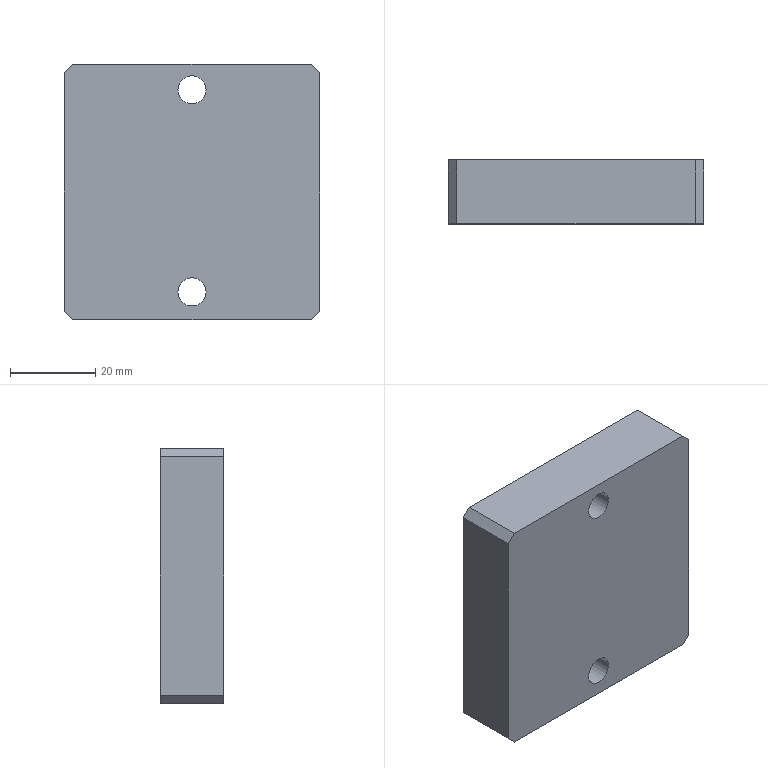Component | SolidWorks | CHEN123-AA-08-1 | 1 solid | 20 faces | box 60 x 15 x 60 mm | volume 52075 mm3 | plane 12 | cylinder 8 | commonest cylinder face diameters 11 x4 6.6 x4
build123d program:
from build123d import *

# Parameters (mm, degrees)
SKETCH1_W                                       = 60
SKETCH1_H                                       = 60
BOSS_EXTRUDE1_DEPTH                             = 15
CHAMFER1_SIZE                                   = 2
M6_HEX_SOCKET_HEAD_CAP_SCREW_CBORE1_D           = 6.6
M6_HEX_SOCKET_HEAD_CAP_SCREW_CBORE1_CBORE_D     = 11
M6_HEX_SOCKET_HEAD_CAP_SCREW_CBORE1_CBORE_DEPTH = 6.4


with BuildPart() as part:
    # Sketch1 → Boss-Extrude1 (new body)
    with BuildSketch(Plane.XY):
        Rectangle(SKETCH1_W, SKETCH1_H)
    extrude(amount=BOSS_EXTRUDE1_DEPTH)

    # Chamfer1
    chamfer1_edges = [part.edges().sort_by_distance(p)[0] for p in [
        (30, -30, 7.5),
        (-30, -30, 7.5),
        (-30, 30, 7.5),
        (30, 30, 7.5),
    ]]
    chamfer(chamfer1_edges, length=CHAMFER1_SIZE)

    # M6 Hex Socket Head Cap Screw CBORE1 (through all)
    with Locations(Plane.XY.offset(15)):
        with Locations((0, 23.473), (0, -23.997)):
            CounterBoreHole(M6_HEX_SOCKET_HEAD_CAP_SCREW_CBORE1_D / 2, M6_HEX_SOCKET_HEAD_CAP_SCREW_CBORE1_CBORE_D / 2, M6_HEX_SOCKET_HEAD_CAP_SCREW_CBORE1_CBORE_DEPTH)


solid = part.part

# Placed as in the assembly
solid = solid.moved(Location((-0.0005, -150.999, -97), (-90, 0, 0)))
STEP:
#1=CARTESIAN_POINT('',(-0.2166,-5.606,-4.743));
#2=VERTEX_POINT('',#1);
#3=CARTESIAN_POINT('',(0.2165,-5.606,-4.743));
#4=VERTEX_POINT('',#3);
#5=CARTESIAN_POINT('',(-0.00001969,-5.606,-4.743));
#6=DIRECTION('',(0.,1.,0.));
#7=DIRECTION('',(1.,0.,0.));
#8=AXIS2_PLACEMENT_3D('',#5,#6,#7);
#9=CIRCLE('',#8,0.2165);
#10=EDGE_CURVE('',#2,#4,#9,.T.);
#11=ORIENTED_EDGE('',*,*,#10,.F.);
#12=CARTESIAN_POINT('',(-0.2166,-5.354,-4.743));
#13=VERTEX_POINT('',#12);
#14=CARTESIAN_POINT('',(-0.2166,-5.354,-4.743));
#15=DIRECTION('',(0.,1.,0.));
#16=VECTOR('',#15,39.37);
#17=LINE('',#14,#16);
#18=EDGE_CURVE('',#2,#13,#17,.T.);
#19=ORIENTED_EDGE('',*,*,#18,.T.);
#20=CARTESIAN_POINT('',(0.2165,-5.354,-4.743));
#21=VERTEX_POINT('',#20);
#22=CARTESIAN_POINT('',(-0.00001969,-5.354,-4.743));
#23=DIRECTION('',(0.,1.,0.));
#24=DIRECTION('',(1.,0.,0.));
#25=AXIS2_PLACEMENT_3D('',#22,#23,#24);
#26=CIRCLE('',#25,0.2165);
#27=EDGE_CURVE('',#13,#21,#26,.T.);
#28=ORIENTED_EDGE('',*,*,#27,.T.);
#29=CARTESIAN_POINT('',(0.2165,-5.354,-4.743));
#30=DIRECTION('',(0.,1.,0.));
#31=VECTOR('',#30,39.37);
#32=LINE('',#29,#31);
#33=EDGE_CURVE('',#4,#21,#32,.T.);
#34=ORIENTED_EDGE('',*,*,#33,.F.);
#35=EDGE_LOOP('',(#11,#19,#28,#34));
#36=FACE_OUTER_BOUND('',#35,.T.);
#37=CARTESIAN_POINT('',(-0.00001969,-5.354,-4.743));
#38=DIRECTION('',(0.,1.,0.));
#39=DIRECTION('',(1.,0.,0.));
#40=AXIS2_PLACEMENT_3D('',#37,#38,#39);
#41=CYLINDRICAL_SURFACE('',#40,0.2165);
#42=ADVANCED_FACE('',(#36),#41,.F.);
#43=CARTESIAN_POINT('',(-0.1299,-5.945,-4.743));
#44=VERTEX_POINT('',#43);
#45=CARTESIAN_POINT('',(0.1299,-5.945,-4.743));
#46=VERTEX_POINT('',#45);
#47=CARTESIAN_POINT('',(-0.00001969,-5.945,-4.743));
#48=DIRECTION('',(0.,1.,0.));
#49=DIRECTION('',(1.,0.,0.));
#50=AXIS2_PLACEMENT_3D('',#47,#48,#49);
#51=CIRCLE('',#50,0.1299);
#52=EDGE_CURVE('',#44,#46,#51,.T.);
#53=ORIENTED_EDGE('',*,*,#52,.F.);
#54=CARTESIAN_POINT('',(-0.1299,-5.606,-4.743));
#55=VERTEX_POINT('',#54);
#56=CARTESIAN_POINT('',(-0.1299,-5.354,-4.743));
#57=DIRECTION('',(0.,1.,0.));
#58=VECTOR('',#57,39.37);
#59=LINE('',#56,#58);
#60=EDGE_CURVE('',#44,#55,#59,.T.);
#61=ORIENTED_EDGE('',*,*,#60,.T.);
#62=CARTESIAN_POINT('',(0.1299,-5.606,-4.743));
#63=VERTEX_POINT('',#62);
#64=CARTESIAN_POINT('',(-0.00001969,-5.606,-4.743));
#65=DIRECTION('',(0.,1.,0.));
#66=DIRECTION('',(1.,0.,0.));
#67=AXIS2_PLACEMENT_3D('',#64,#65,#66);
#68=CIRCLE('',#67,0.1299);
#69=EDGE_CURVE('',#55,#63,#68,.T.);
#70=ORIENTED_EDGE('',*,*,#69,.T.);
#71=CARTESIAN_POINT('',(0.1299,-5.354,-4.743));
#72=DIRECTION('',(0.,1.,0.));
#73=VECTOR('',#72,39.37);
#74=LINE('',#71,#73);
#75=EDGE_CURVE('',#46,#63,#74,.T.);
#76=ORIENTED_EDGE('',*,*,#75,.F.);
#77=EDGE_LOOP('',(#53,#61,#70,#76));
#78=FACE_OUTER_BOUND('',#77,.T.);
#79=CARTESIAN_POINT('',(-0.00001969,-5.354,-4.743));
#80=DIRECTION('',(0.,1.,0.));
#81=DIRECTION('',(1.,0.,0.));
#82=AXIS2_PLACEMENT_3D('',#79,#80,#81);
#83=CYLINDRICAL_SURFACE('',#82,0.1299);
#84=ADVANCED_FACE('',(#78),#83,.F.);
#85=CARTESIAN_POINT('',(-0.2166,-5.606,-2.874));
#86=VERTEX_POINT('',#85);
#87=CARTESIAN_POINT('',(0.2165,-5.606,-2.874));
#88=VERTEX_POINT('',#87);
#89=CARTESIAN_POINT('',(-0.00001969,-5.606,-2.874));
#90=DIRECTION('',(0.,1.,0.));
#91=DIRECTION('',(1.,0.,0.));
#92=AXIS2_PLACEMENT_3D('',#89,#90,#91);
#93=CIRCLE('',#92,0.2165);
#94=EDGE_CURVE('',#86,#88,#93,.T.);
#95=ORIENTED_EDGE('',*,*,#94,.F.);
#96=CARTESIAN_POINT('',(-0.2166,-5.354,-2.874));
#97=VERTEX_POINT('',#96);
#98=CARTESIAN_POINT('',(-0.2166,-5.354,-2.874));
#99=DIRECTION('',(0.,1.,0.));
#100=VECTOR('',#99,39.37);
#101=LINE('',#98,#100);
#102=EDGE_CURVE('',#86,#97,#101,.T.);
#103=ORIENTED_EDGE('',*,*,#102,.T.);
#104=CARTESIAN_POINT('',(0.2165,-5.354,-2.874));
#105=VERTEX_POINT('',#104);
#106=CARTESIAN_POINT('',(-0.00001969,-5.354,-2.874));
#107=DIRECTION('',(0.,1.,0.));
#108=DIRECTION('',(1.,0.,0.));
#109=AXIS2_PLACEMENT_3D('',#106,#107,#108);
#110=CIRCLE('',#109,0.2165);
#111=EDGE_CURVE('',#97,#105,#110,.T.);
#112=ORIENTED_EDGE('',*,*,#111,.T.);
#113=CARTESIAN_POINT('',(0.2165,-5.354,-2.874));
#114=DIRECTION('',(0.,1.,0.));
#115=VECTOR('',#114,39.37);
#116=LINE('',#113,#115);
#117=EDGE_CURVE('',#88,#105,#116,.T.);
#118=ORIENTED_EDGE('',*,*,#117,.F.);
#119=EDGE_LOOP('',(#95,#103,#112,#118));
#120=FACE_OUTER_BOUND('',#119,.T.);
#121=CARTESIAN_POINT('',(-0.00001969,-5.354,-2.874));
#122=DIRECTION('',(0.,1.,0.));
#123=DIRECTION('',(1.,0.,0.));
#124=AXIS2_PLACEMENT_3D('',#121,#122,#123);
#125=CYLINDRICAL_SURFACE('',#124,0.2165);
#126=ADVANCED_FACE('',(#120),#125,.F.);
#127=CARTESIAN_POINT('',(-0.1299,-5.945,-2.874));
#128=VERTEX_POINT('',#127);
#129=CARTESIAN_POINT('',(0.1299,-5.945,-2.874));
#130=VERTEX_POINT('',#129);
#131=CARTESIAN_POINT('',(-0.00001969,-5.945,-2.874));
#132=DIRECTION('',(0.,1.,0.));
#133=DIRECTION('',(1.,0.,0.));
#134=AXIS2_PLACEMENT_3D('',#131,#132,#133);
#135=CIRCLE('',#134,0.1299);
#136=EDGE_CURVE('',#128,#130,#135,.T.);
#137=ORIENTED_EDGE('',*,*,#136,.F.);
#138=CARTESIAN_POINT('',(-0.1299,-5.606,-2.874));
#139=VERTEX_POINT('',#138);
#140=CARTESIAN_POINT('',(-0.1299,-5.354,-2.874));
#141=DIRECTION('',(0.,1.,0.));
#142=VECTOR('',#141,39.37);
#143=LINE('',#140,#142);
#144=EDGE_CURVE('',#128,#139,#143,.T.);
#145=ORIENTED_EDGE('',*,*,#144,.T.);
#146=CARTESIAN_POINT('',(0.1299,-5.606,-2.874));
#147=VERTEX_POINT('',#146);
#148=CARTESIAN_POINT('',(-0.00001969,-5.606,-2.874));
#149=DIRECTION('',(0.,1.,0.));
#150=DIRECTION('',(1.,0.,0.));
#151=AXIS2_PLACEMENT_3D('',#148,#149,#150);
#152=CIRCLE('',#151,0.1299);
#153=EDGE_CURVE('',#139,#147,#152,.T.);
#154=ORIENTED_EDGE('',*,*,#153,.T.);
#155=CARTESIAN_POINT('',(0.1299,-5.354,-2.874));
#156=DIRECTION('',(0.,1.,0.));
#157=VECTOR('',#156,39.37);
#158=LINE('',#155,#157);
#159=EDGE_CURVE('',#130,#147,#158,.T.);
#160=ORIENTED_EDGE('',*,*,#159,.F.);
#161=EDGE_LOOP('',(#137,#145,#154,#160));
#162=FACE_OUTER_BOUND('',#161,.T.);
#163=CARTESIAN_POINT('',(-0.00001969,-5.354,-2.874));
#164=DIRECTION('',(0.,1.,0.));
#165=DIRECTION('',(1.,0.,0.));
#166=AXIS2_PLACEMENT_3D('',#163,#164,#165);
#167=CYLINDRICAL_SURFACE('',#166,0.1299);
#168=ADVANCED_FACE('',(#162),#167,.F.);
#169=CARTESIAN_POINT('',(1.181,-5.354,-2.717));
#170=VERTEX_POINT('',#169);
#171=CARTESIAN_POINT('',(1.181,-5.354,-4.921));
#172=VERTEX_POINT('',#171);
#173=CARTESIAN_POINT('',(1.181,-5.354,-2.638));
#174=DIRECTION('',(0.,0.,-1.));
#175=VECTOR('',#174,39.37);
#176=LINE('',#173,#175);
#177=EDGE_CURVE('',#170,#172,#176,.T.);
#178=ORIENTED_EDGE('',*,*,#177,.F.);
#179=CARTESIAN_POINT('',(1.181,-5.945,-2.717));
#180=VERTEX_POINT('',#179);
#181=CARTESIAN_POINT('',(1.181,-5.354,-2.717));
#182=DIRECTION('',(0.,-1.,0.));
#183=VECTOR('',#182,39.37);
#184=LINE('',#181,#183);
#185=EDGE_CURVE('',#170,#180,#184,.T.);
#186=ORIENTED_EDGE('',*,*,#185,.T.);
#187=CARTESIAN_POINT('',(1.181,-5.945,-4.921));
#188=VERTEX_POINT('',#187);
#189=CARTESIAN_POINT('',(1.181,-5.945,-2.638));
#190=DIRECTION('',(0.,0.,-1.));
#191=VECTOR('',#190,39.37);
#192=LINE('',#189,#191);
#193=EDGE_CURVE('',#180,#188,#192,.T.);
#194=ORIENTED_EDGE('',*,*,#193,.T.);
#195=CARTESIAN_POINT('',(1.181,-5.354,-4.921));
#196=DIRECTION('',(0.,1.,0.));
#197=VECTOR('',#196,39.37);
#198=LINE('',#195,#197);
#199=EDGE_CURVE('',#188,#172,#198,.T.);
#200=ORIENTED_EDGE('',*,*,#199,.T.);
#201=EDGE_LOOP('',(#178,#186,#194,#200));
#202=FACE_OUTER_BOUND('',#201,.T.);
#203=CARTESIAN_POINT('',(1.181,-5.354,-2.638));
#204=DIRECTION('',(-1.,0.,0.));
#205=DIRECTION('',(0.,1.,0.));
#206=AXIS2_PLACEMENT_3D('',#203,#204,#205);
#207=PLANE('',#206);
#208=ADVANCED_FACE('',(#202),#207,.F.);
#209=CARTESIAN_POINT('',(1.102,-5.354,-5.));
#210=VERTEX_POINT('',#209);
#211=CARTESIAN_POINT('',(-1.102,-5.354,-5.));
#212=VERTEX_POINT('',#211);
#213=CARTESIAN_POINT('',(-1.181,-5.354,-5.));
#214=DIRECTION('',(-1.,0.,0.));
#215=VECTOR('',#214,39.37);
#216=LINE('',#213,#215);
#217=EDGE_CURVE('',#210,#212,#216,.T.);
#218=ORIENTED_EDGE('',*,*,#217,.F.);
#219=CARTESIAN_POINT('',(1.102,-5.945,-5.));
#220=VERTEX_POINT('',#219);
#221=CARTESIAN_POINT('',(1.102,-5.354,-5.));
#222=DIRECTION('',(0.,-1.,0.));
#223=VECTOR('',#222,39.37);
#224=LINE('',#221,#223);
#225=EDGE_CURVE('',#210,#220,#224,.T.);
#226=ORIENTED_EDGE('',*,*,#225,.T.);
#227=CARTESIAN_POINT('',(-1.102,-5.945,-5.));
#228=VERTEX_POINT('',#227);
#229=CARTESIAN_POINT('',(-1.181,-5.945,-5.));
#230=DIRECTION('',(-1.,0.,0.));
#231=VECTOR('',#230,39.37);
#232=LINE('',#229,#231);
#233=EDGE_CURVE('',#220,#228,#232,.T.);
#234=ORIENTED_EDGE('',*,*,#233,.T.);
#235=CARTESIAN_POINT('',(-1.102,-5.354,-5.));
#236=DIRECTION('',(0.,1.,0.));
#237=VECTOR('',#236,39.37);
#238=LINE('',#235,#237);
#239=EDGE_CURVE('',#228,#212,#238,.T.);
#240=ORIENTED_EDGE('',*,*,#239,.T.);
#241=EDGE_LOOP('',(#218,#226,#234,#240));
#242=FACE_OUTER_BOUND('',#241,.T.);
#243=CARTESIAN_POINT('',(-1.181,-5.354,-5.));
#244=DIRECTION('',(0.,0.,1.));
#245=DIRECTION('',(0.,-1.,0.));
#246=AXIS2_PLACEMENT_3D('',#243,#244,#245);
#247=PLANE('',#246);
#248=ADVANCED_FACE('',(#242),#247,.F.);
#249=CARTESIAN_POINT('',(-1.181,-5.945,-4.921));
#250=VERTEX_POINT('',#249);
#251=CARTESIAN_POINT('',(-1.181,-5.945,-2.717));
#252=VERTEX_POINT('',#251);
#253=CARTESIAN_POINT('',(-1.181,-5.945,-2.638));
#254=DIRECTION('',(0.,0.,1.));
#255=VECTOR('',#254,39.37);
#256=LINE('',#253,#255);
#257=EDGE_CURVE('',#250,#252,#256,.T.);
#258=ORIENTED_EDGE('',*,*,#257,.T.);
#259=CARTESIAN_POINT('',(-1.181,-5.354,-2.717));
#260=VERTEX_POINT('',#259);
#261=CARTESIAN_POINT('',(-1.181,-5.354,-2.717));
#262=DIRECTION('',(0.,1.,0.));
#263=VECTOR('',#262,39.37);
#264=LINE('',#261,#263);
#265=EDGE_CURVE('',#252,#260,#264,.T.);
#266=ORIENTED_EDGE('',*,*,#265,.T.);
#267=CARTESIAN_POINT('',(-1.181,-5.354,-4.921));
#268=VERTEX_POINT('',#267);
#269=CARTESIAN_POINT('',(-1.181,-5.354,-2.638));
#270=DIRECTION('',(0.,0.,1.));
#271=VECTOR('',#270,39.37);
#272=LINE('',#269,#271);
#273=EDGE_CURVE('',#268,#260,#272,.T.);
#274=ORIENTED_EDGE('',*,*,#273,.F.);
#275=CARTESIAN_POINT('',(-1.181,-5.354,-4.921));
#276=DIRECTION('',(0.,-1.,0.));
#277=VECTOR('',#276,39.37);
#278=LINE('',#275,#277);
#279=EDGE_CURVE('',#268,#250,#278,.T.);
#280=ORIENTED_EDGE('',*,*,#279,.T.);
#281=EDGE_LOOP('',(#258,#266,#274,#280));
#282=FACE_OUTER_BOUND('',#281,.T.);
#283=CARTESIAN_POINT('',(-1.181,-5.354,-2.638));
#284=DIRECTION('',(1.,0.,0.));
#285=DIRECTION('',(0.,-1.,0.));
#286=AXIS2_PLACEMENT_3D('',#283,#284,#285);
#287=PLANE('',#286);
#288=ADVANCED_FACE('',(#282),#287,.F.);
#289=CARTESIAN_POINT('',(-1.102,-5.945,-2.638));
#290=VERTEX_POINT('',#289);
#291=CARTESIAN_POINT('',(1.102,-5.945,-2.638));
#292=VERTEX_POINT('',#291);
#293=CARTESIAN_POINT('',(-1.181,-5.945,-2.638));
#294=DIRECTION('',(1.,0.,0.));
#295=VECTOR('',#294,39.37);
#296=LINE('',#293,#295);
#297=EDGE_CURVE('',#290,#292,#296,.T.);
#298=ORIENTED_EDGE('',*,*,#297,.T.);
#299=CARTESIAN_POINT('',(1.102,-5.354,-2.638));
#300=VERTEX_POINT('',#299);
#301=CARTESIAN_POINT('',(1.102,-5.354,-2.638));
#302=DIRECTION('',(0.,1.,0.));
#303=VECTOR('',#302,39.37);
#304=LINE('',#301,#303);
#305=EDGE_CURVE('',#292,#300,#304,.T.);
#306=ORIENTED_EDGE('',*,*,#305,.T.);
#307=CARTESIAN_POINT('',(-1.102,-5.354,-2.638));
#308=VERTEX_POINT('',#307);
#309=CARTESIAN_POINT('',(-1.181,-5.354,-2.638));
#310=DIRECTION('',(1.,0.,0.));
#311=VECTOR('',#310,39.37);
#312=LINE('',#309,#311);
#313=EDGE_CURVE('',#308,#300,#312,.T.);
#314=ORIENTED_EDGE('',*,*,#313,.F.);
#315=CARTESIAN_POINT('',(-1.102,-5.354,-2.638));
#316=DIRECTION('',(0.,-1.,0.));
#317=VECTOR('',#316,39.37);
#318=LINE('',#315,#317);
#319=EDGE_CURVE('',#308,#290,#318,.T.);
#320=ORIENTED_EDGE('',*,*,#319,.T.);
#321=EDGE_LOOP('',(#298,#306,#314,#320));
#322=FACE_OUTER_BOUND('',#321,.T.);
#323=CARTESIAN_POINT('',(-1.181,-5.354,-2.638));
#324=DIRECTION('',(0.,0.,-1.));
#325=DIRECTION('',(0.,1.,0.));
#326=AXIS2_PLACEMENT_3D('',#323,#324,#325);
#327=PLANE('',#326);
#328=ADVANCED_FACE('',(#322),#327,.F.);
#329=CARTESIAN_POINT('',(-0.00001969,-5.354,-4.743));
#330=DIRECTION('',(0.,1.,0.));
#331=DIRECTION('',(1.,0.,0.));
#332=AXIS2_PLACEMENT_3D('',#329,#330,#331);
#333=CIRCLE('',#332,0.2165);
#334=EDGE_CURVE('',#21,#13,#333,.T.);
#335=ORIENTED_EDGE('',*,*,#334,.F.);
#336=ORIENTED_EDGE('',*,*,#27,.F.);
#337=EDGE_LOOP('',(#335,#336));
#338=FACE_BOUND('',#337,.T.);
#339=CARTESIAN_POINT('',(-0.00001969,-5.354,-2.874));
#340=DIRECTION('',(0.,1.,0.));
#341=DIRECTION('',(1.,0.,0.));
#342=AXIS2_PLACEMENT_3D('',#339,#340,#341);
#343=CIRCLE('',#342,0.2165);
#344=EDGE_CURVE('',#105,#97,#343,.T.);
#345=ORIENTED_EDGE('',*,*,#344,.F.);
#346=ORIENTED_EDGE('',*,*,#111,.F.);
#347=EDGE_LOOP('',(#345,#346));
#348=FACE_BOUND('',#347,.T.);
#349=ORIENTED_EDGE('',*,*,#313,.T.);
#350=CARTESIAN_POINT('',(1.181,-5.354,-2.717));
#351=DIRECTION('',(0.7071,0.,-0.7071));
#352=VECTOR('',#351,39.37);
#353=LINE('',#350,#352);
#354=EDGE_CURVE('',#300,#170,#353,.T.);
#355=ORIENTED_EDGE('',*,*,#354,.T.);
#356=ORIENTED_EDGE('',*,*,#177,.T.);
#357=CARTESIAN_POINT('',(1.102,-5.354,-5.));
#358=DIRECTION('',(-0.7071,0.,-0.7071));
#359=VECTOR('',#358,39.37);
#360=LINE('',#357,#359);
#361=EDGE_CURVE('',#172,#210,#360,.T.);
#362=ORIENTED_EDGE('',*,*,#361,.T.);
#363=ORIENTED_EDGE('',*,*,#217,.T.);
#364=CARTESIAN_POINT('',(-1.181,-5.354,-4.921));
#365=DIRECTION('',(-0.7071,0.,0.7071));
#366=VECTOR('',#365,39.37);
#367=LINE('',#364,#366);
#368=EDGE_CURVE('',#212,#268,#367,.T.);
#369=ORIENTED_EDGE('',*,*,#368,.T.);
#370=ORIENTED_EDGE('',*,*,#273,.T.);
#371=CARTESIAN_POINT('',(-1.102,-5.354,-2.638));
#372=DIRECTION('',(0.7071,0.,0.7071));
#373=VECTOR('',#372,39.37);
#374=LINE('',#371,#373);
#375=EDGE_CURVE('',#260,#308,#374,.T.);
#376=ORIENTED_EDGE('',*,*,#375,.T.);
#377=EDGE_LOOP('',(#349,#355,#356,#362,#363,#369,#370,#376));
#378=FACE_OUTER_BOUND('',#377,.T.);
#379=CARTESIAN_POINT('',(-0.00001969,-5.354,-3.819));
#380=DIRECTION('',(0.,-1.,0.));
#381=DIRECTION('',(-1.,0.,0.));
#382=AXIS2_PLACEMENT_3D('',#379,#380,#381);
#383=PLANE('',#382);
#384=ADVANCED_FACE('',(#338,#348,#378),#383,.F.);
#385=CARTESIAN_POINT('',(-0.00001969,-5.945,-4.743));
#386=DIRECTION('',(0.,1.,0.));
#387=DIRECTION('',(1.,0.,0.));
#388=AXIS2_PLACEMENT_3D('',#385,#386,#387);
#389=CIRCLE('',#388,0.1299);
#390=EDGE_CURVE('',#46,#44,#389,.T.);
#391=ORIENTED_EDGE('',*,*,#390,.T.);
#392=ORIENTED_EDGE('',*,*,#52,.T.);
#393=EDGE_LOOP('',(#391,#392));
#394=FACE_BOUND('',#393,.T.);
#395=CARTESIAN_POINT('',(-0.00001969,-5.945,-2.874));
#396=DIRECTION('',(0.,1.,0.));
#397=DIRECTION('',(1.,0.,0.));
#398=AXIS2_PLACEMENT_3D('',#395,#396,#397);
#399=CIRCLE('',#398,0.1299);
#400=EDGE_CURVE('',#130,#128,#399,.T.);
#401=ORIENTED_EDGE('',*,*,#400,.T.);
#402=ORIENTED_EDGE('',*,*,#136,.T.);
#403=EDGE_LOOP('',(#401,#402));
#404=FACE_BOUND('',#403,.T.);
#405=ORIENTED_EDGE('',*,*,#193,.F.);
#406=CARTESIAN_POINT('',(1.142,-5.945,-2.677));
#407=DIRECTION('',(-0.7071,0.,0.7071));
#408=VECTOR('',#407,39.37);
#409=LINE('',#406,#408);
#410=EDGE_CURVE('',#180,#292,#409,.T.);
#411=ORIENTED_EDGE('',*,*,#410,.T.);
#412=ORIENTED_EDGE('',*,*,#297,.F.);
#413=CARTESIAN_POINT('',(-1.142,-5.945,-2.677));
#414=DIRECTION('',(-0.7071,0.,-0.7071));
#415=VECTOR('',#414,39.37);
#416=LINE('',#413,#415);
#417=EDGE_CURVE('',#290,#252,#416,.T.);
#418=ORIENTED_EDGE('',*,*,#417,.T.);
#419=ORIENTED_EDGE('',*,*,#257,.F.);
#420=CARTESIAN_POINT('',(-1.142,-5.945,-4.961));
#421=DIRECTION('',(0.7071,0.,-0.7071));
#422=VECTOR('',#421,39.37);
#423=LINE('',#420,#422);
#424=EDGE_CURVE('',#250,#228,#423,.T.);
#425=ORIENTED_EDGE('',*,*,#424,.T.);
#426=ORIENTED_EDGE('',*,*,#233,.F.);
#427=CARTESIAN_POINT('',(1.142,-5.945,-4.961));
#428=DIRECTION('',(0.7071,0.,0.7071));
#429=VECTOR('',#428,39.37);
#430=LINE('',#427,#429);
#431=EDGE_CURVE('',#220,#188,#430,.T.);
#432=ORIENTED_EDGE('',*,*,#431,.T.);
#433=EDGE_LOOP('',(#405,#411,#412,#418,#419,#425,#426,#432));
#434=FACE_OUTER_BOUND('',#433,.T.);
#435=CARTESIAN_POINT('',(-0.00001969,-5.945,-3.819));
#436=DIRECTION('',(0.,-1.,0.));
#437=DIRECTION('',(-1.,0.,0.));
#438=AXIS2_PLACEMENT_3D('',#435,#436,#437);
#439=PLANE('',#438);
#440=ADVANCED_FACE('',(#394,#404,#434),#439,.T.);
#441=ORIENTED_EDGE('',*,*,#354,.F.);
#442=ORIENTED_EDGE('',*,*,#305,.F.);
#443=ORIENTED_EDGE('',*,*,#410,.F.);
#444=ORIENTED_EDGE('',*,*,#185,.F.);
#445=EDGE_LOOP('',(#441,#442,#443,#444));
#446=FACE_OUTER_BOUND('',#445,.T.);
#447=CARTESIAN_POINT('',(1.181,-5.354,-2.717));
#448=DIRECTION('',(-0.7071,0.,-0.7071));
#449=DIRECTION('',(0.,-1.,0.));
#450=AXIS2_PLACEMENT_3D('',#447,#448,#449);
#451=PLANE('',#450);
#452=ADVANCED_FACE('',(#446),#451,.F.);
#453=ORIENTED_EDGE('',*,*,#375,.F.);
#454=ORIENTED_EDGE('',*,*,#265,.F.);
#455=ORIENTED_EDGE('',*,*,#417,.F.);
#456=ORIENTED_EDGE('',*,*,#319,.F.);
#457=EDGE_LOOP('',(#453,#454,#455,#456));
#458=FACE_OUTER_BOUND('',#457,.T.);
#459=CARTESIAN_POINT('',(-1.102,-5.354,-2.638));
#460=DIRECTION('',(0.7071,0.,-0.7071));
#461=DIRECTION('',(0.,-1.,0.));
#462=AXIS2_PLACEMENT_3D('',#459,#460,#461);
#463=PLANE('',#462);
#464=ADVANCED_FACE('',(#458),#463,.F.);
#465=ORIENTED_EDGE('',*,*,#361,.F.);
#466=ORIENTED_EDGE('',*,*,#199,.F.);
#467=ORIENTED_EDGE('',*,*,#431,.F.);
#468=ORIENTED_EDGE('',*,*,#225,.F.);
#469=EDGE_LOOP('',(#465,#466,#467,#468));
#470=FACE_OUTER_BOUND('',#469,.T.);
#471=CARTESIAN_POINT('',(1.102,-5.354,-5.));
#472=DIRECTION('',(-0.7071,0.,0.7071));
#473=DIRECTION('',(0.,-1.,0.));
#474=AXIS2_PLACEMENT_3D('',#471,#472,#473);
#475=PLANE('',#474);
#476=ADVANCED_FACE('',(#470),#475,.F.);
#477=ORIENTED_EDGE('',*,*,#368,.F.);
#478=ORIENTED_EDGE('',*,*,#239,.F.);
#479=ORIENTED_EDGE('',*,*,#424,.F.);
#480=ORIENTED_EDGE('',*,*,#279,.F.);
#481=EDGE_LOOP('',(#477,#478,#479,#480));
#482=FACE_OUTER_BOUND('',#481,.T.);
#483=CARTESIAN_POINT('',(-1.181,-5.354,-4.921));
#484=DIRECTION('',(0.7071,0.,0.7071));
#485=DIRECTION('',(0.,-1.,0.));
#486=AXIS2_PLACEMENT_3D('',#483,#484,#485);
#487=PLANE('',#486);
#488=ADVANCED_FACE('',(#482),#487,.F.);
#489=ORIENTED_EDGE('',*,*,#144,.F.);
#490=ORIENTED_EDGE('',*,*,#400,.F.);
#491=ORIENTED_EDGE('',*,*,#159,.T.);
#492=CARTESIAN_POINT('',(-0.00001969,-5.606,-2.874));
#493=DIRECTION('',(0.,1.,0.));
#494=DIRECTION('',(1.,0.,0.));
#495=AXIS2_PLACEMENT_3D('',#492,#493,#494);
#496=CIRCLE('',#495,0.1299);
#497=EDGE_CURVE('',#147,#139,#496,.T.);
#498=ORIENTED_EDGE('',*,*,#497,.T.);
#499=EDGE_LOOP('',(#489,#490,#491,#498));
#500=FACE_OUTER_BOUND('',#499,.T.);
#501=CARTESIAN_POINT('',(-0.00001969,-5.354,-2.874));
#502=DIRECTION('',(0.,1.,0.));
#503=DIRECTION('',(1.,0.,0.));
#504=AXIS2_PLACEMENT_3D('',#501,#502,#503);
#505=CYLINDRICAL_SURFACE('',#504,0.1299);
#506=ADVANCED_FACE('',(#500),#505,.F.);
#507=ORIENTED_EDGE('',*,*,#497,.F.);
#508=ORIENTED_EDGE('',*,*,#153,.F.);
#509=EDGE_LOOP('',(#507,#508));
#510=FACE_BOUND('',#509,.T.);
#511=CARTESIAN_POINT('',(-0.00001969,-5.606,-2.874));
#512=DIRECTION('',(0.,1.,0.));
#513=DIRECTION('',(1.,0.,0.));
#514=AXIS2_PLACEMENT_3D('',#511,#512,#513);
#515=CIRCLE('',#514,0.2165);
#516=EDGE_CURVE('',#88,#86,#515,.T.);
#517=ORIENTED_EDGE('',*,*,#516,.T.);
#518=ORIENTED_EDGE('',*,*,#94,.T.);
#519=EDGE_LOOP('',(#517,#518));
#520=FACE_OUTER_BOUND('',#519,.T.);
#521=CARTESIAN_POINT('',(0.1299,-5.606,-2.874));
#522=DIRECTION('',(0.,-1.,0.));
#523=DIRECTION('',(-1.,0.,0.));
#524=AXIS2_PLACEMENT_3D('',#521,#522,#523);
#525=PLANE('',#524);
#526=ADVANCED_FACE('',(#510,#520),#525,.F.);
#527=ORIENTED_EDGE('',*,*,#102,.F.);
#528=ORIENTED_EDGE('',*,*,#516,.F.);
#529=ORIENTED_EDGE('',*,*,#117,.T.);
#530=ORIENTED_EDGE('',*,*,#344,.T.);
#531=EDGE_LOOP('',(#527,#528,#529,#530));
#532=FACE_OUTER_BOUND('',#531,.T.);
#533=CARTESIAN_POINT('',(-0.00001969,-5.354,-2.874));
#534=DIRECTION('',(0.,1.,0.));
#535=DIRECTION('',(1.,0.,0.));
#536=AXIS2_PLACEMENT_3D('',#533,#534,#535);
#537=CYLINDRICAL_SURFACE('',#536,0.2165);
#538=ADVANCED_FACE('',(#532),#537,.F.);
#539=ORIENTED_EDGE('',*,*,#60,.F.);
#540=ORIENTED_EDGE('',*,*,#390,.F.);
#541=ORIENTED_EDGE('',*,*,#75,.T.);
#542=CARTESIAN_POINT('',(-0.00001969,-5.606,-4.743));
#543=DIRECTION('',(0.,1.,0.));
#544=DIRECTION('',(1.,0.,0.));
#545=AXIS2_PLACEMENT_3D('',#542,#543,#544);
#546=CIRCLE('',#545,0.1299);
#547=EDGE_CURVE('',#63,#55,#546,.T.);
#548=ORIENTED_EDGE('',*,*,#547,.T.);
#549=EDGE_LOOP('',(#539,#540,#541,#548));
#550=FACE_OUTER_BOUND('',#549,.T.);
#551=CARTESIAN_POINT('',(-0.00001969,-5.354,-4.743));
#552=DIRECTION('',(0.,1.,0.));
#553=DIRECTION('',(1.,0.,0.));
#554=AXIS2_PLACEMENT_3D('',#551,#552,#553);
#555=CYLINDRICAL_SURFACE('',#554,0.1299);
#556=ADVANCED_FACE('',(#550),#555,.F.);
#557=ORIENTED_EDGE('',*,*,#547,.F.);
#558=ORIENTED_EDGE('',*,*,#69,.F.);
#559=EDGE_LOOP('',(#557,#558));
#560=FACE_BOUND('',#559,.T.);
#561=CARTESIAN_POINT('',(-0.00001969,-5.606,-4.743));
#562=DIRECTION('',(0.,1.,0.));
#563=DIRECTION('',(1.,0.,0.));
#564=AXIS2_PLACEMENT_3D('',#561,#562,#563);
#565=CIRCLE('',#564,0.2165);
#566=EDGE_CURVE('',#4,#2,#565,.T.);
#567=ORIENTED_EDGE('',*,*,#566,.T.);
#568=ORIENTED_EDGE('',*,*,#10,.T.);
#569=EDGE_LOOP('',(#567,#568));
#570=FACE_OUTER_BOUND('',#569,.T.);
#571=CARTESIAN_POINT('',(0.1299,-5.606,-4.743));
#572=DIRECTION('',(0.,-1.,0.));
#573=DIRECTION('',(-1.,0.,0.));
#574=AXIS2_PLACEMENT_3D('',#571,#572,#573);
#575=PLANE('',#574);
#576=ADVANCED_FACE('',(#560,#570),#575,.F.);
#577=ORIENTED_EDGE('',*,*,#18,.F.);
#578=ORIENTED_EDGE('',*,*,#566,.F.);
#579=ORIENTED_EDGE('',*,*,#33,.T.);
#580=ORIENTED_EDGE('',*,*,#334,.T.);
#581=EDGE_LOOP('',(#577,#578,#579,#580));
#582=FACE_OUTER_BOUND('',#581,.T.);
#583=CARTESIAN_POINT('',(-0.00001969,-5.354,-4.743));
#584=DIRECTION('',(0.,1.,0.));
#585=DIRECTION('',(1.,0.,0.));
#586=AXIS2_PLACEMENT_3D('',#583,#584,#585);
#587=CYLINDRICAL_SURFACE('',#586,0.2165);
#588=ADVANCED_FACE('',(#582),#587,.F.);
#589=CLOSED_SHELL('',(#42,#84,#126,#168,#208,#248,#288,#328,#384,#440,#452,#464,#476,#488,#506,#526,#538,#556,#576,#588));
#590=MANIFOLD_SOLID_BREP('',#589);
#591=CARTESIAN_POINT('',(0.,0.,0.));
#592=DIRECTION('',(0.,0.,1.));
#593=DIRECTION('',(1.,0.,0.));
#594=AXIS2_PLACEMENT_3D('',#591,#592,#593);
#595=(LENGTH_UNIT()NAMED_UNIT(*)SI_UNIT($,.METRE.));
#596=LENGTH_MEASURE_WITH_UNIT(LENGTH_MEASURE(0.0254),#595);
#597=DIMENSIONAL_EXPONENTS(1.,0.,0.,0.,0.,0.,0.);
#598=(CONVERSION_BASED_UNIT('',#596)LENGTH_UNIT()NAMED_UNIT(#597));
#599=UNCERTAINTY_MEASURE_WITH_UNIT(LENGTH_MEASURE(0.00001),#598,'','');
#600=(NAMED_UNIT(*)PLANE_ANGLE_UNIT()SI_UNIT($,.RADIAN.));
#601=(NAMED_UNIT(*)SI_UNIT($,.STERADIAN.)SOLID_ANGLE_UNIT());
#602=(GEOMETRIC_REPRESENTATION_CONTEXT(3)GLOBAL_UNCERTAINTY_ASSIGNED_CONTEXT((#599))GLOBAL_UNIT_ASSIGNED_CONTEXT((#598,#600,#601))REPRESENTATION_CONTEXT('',''));
#603=ADVANCED_BREP_SHAPE_REPRESENTATION('',(#590,#594),#602);
#604=COLOUR_RGB('',0.7922,0.8196,0.9333);
#605=FILL_AREA_STYLE_COLOUR('',#604);
#606=FILL_AREA_STYLE('',(#605));
#607=SURFACE_STYLE_FILL_AREA(#606);
#608=SURFACE_SIDE_STYLE('',(#607));
#609=SURFACE_STYLE_USAGE(.BOTH.,#608);
#610=PRESENTATION_STYLE_ASSIGNMENT((#609));
#611=STYLED_ITEM('',(#610),#590);
#612=PRESENTATION_LAYER_ASSIGNMENT('','',(#611));
#613=(LENGTH_UNIT()NAMED_UNIT(*)SI_UNIT($,.METRE.));
#614=LENGTH_MEASURE_WITH_UNIT(LENGTH_MEASURE(0.0254),#613);
#615=DIMENSIONAL_EXPONENTS(1.,0.,0.,0.,0.,0.,0.);
#616=(CONVERSION_BASED_UNIT('',#614)LENGTH_UNIT()NAMED_UNIT(#615));
#617=UNCERTAINTY_MEASURE_WITH_UNIT(LENGTH_MEASURE(0.00001),#616,'','');
#618=(NAMED_UNIT(*)PLANE_ANGLE_UNIT()SI_UNIT($,.RADIAN.));
#619=(NAMED_UNIT(*)SI_UNIT($,.STERADIAN.)SOLID_ANGLE_UNIT());
#620=(GEOMETRIC_REPRESENTATION_CONTEXT(3)GLOBAL_UNCERTAINTY_ASSIGNED_CONTEXT((#617))GLOBAL_UNIT_ASSIGNED_CONTEXT((#616,#618,#619))REPRESENTATION_CONTEXT('',''));
#621=MECHANICAL_DESIGN_GEOMETRIC_PRESENTATION_REPRESENTATION('',(#611),#620);